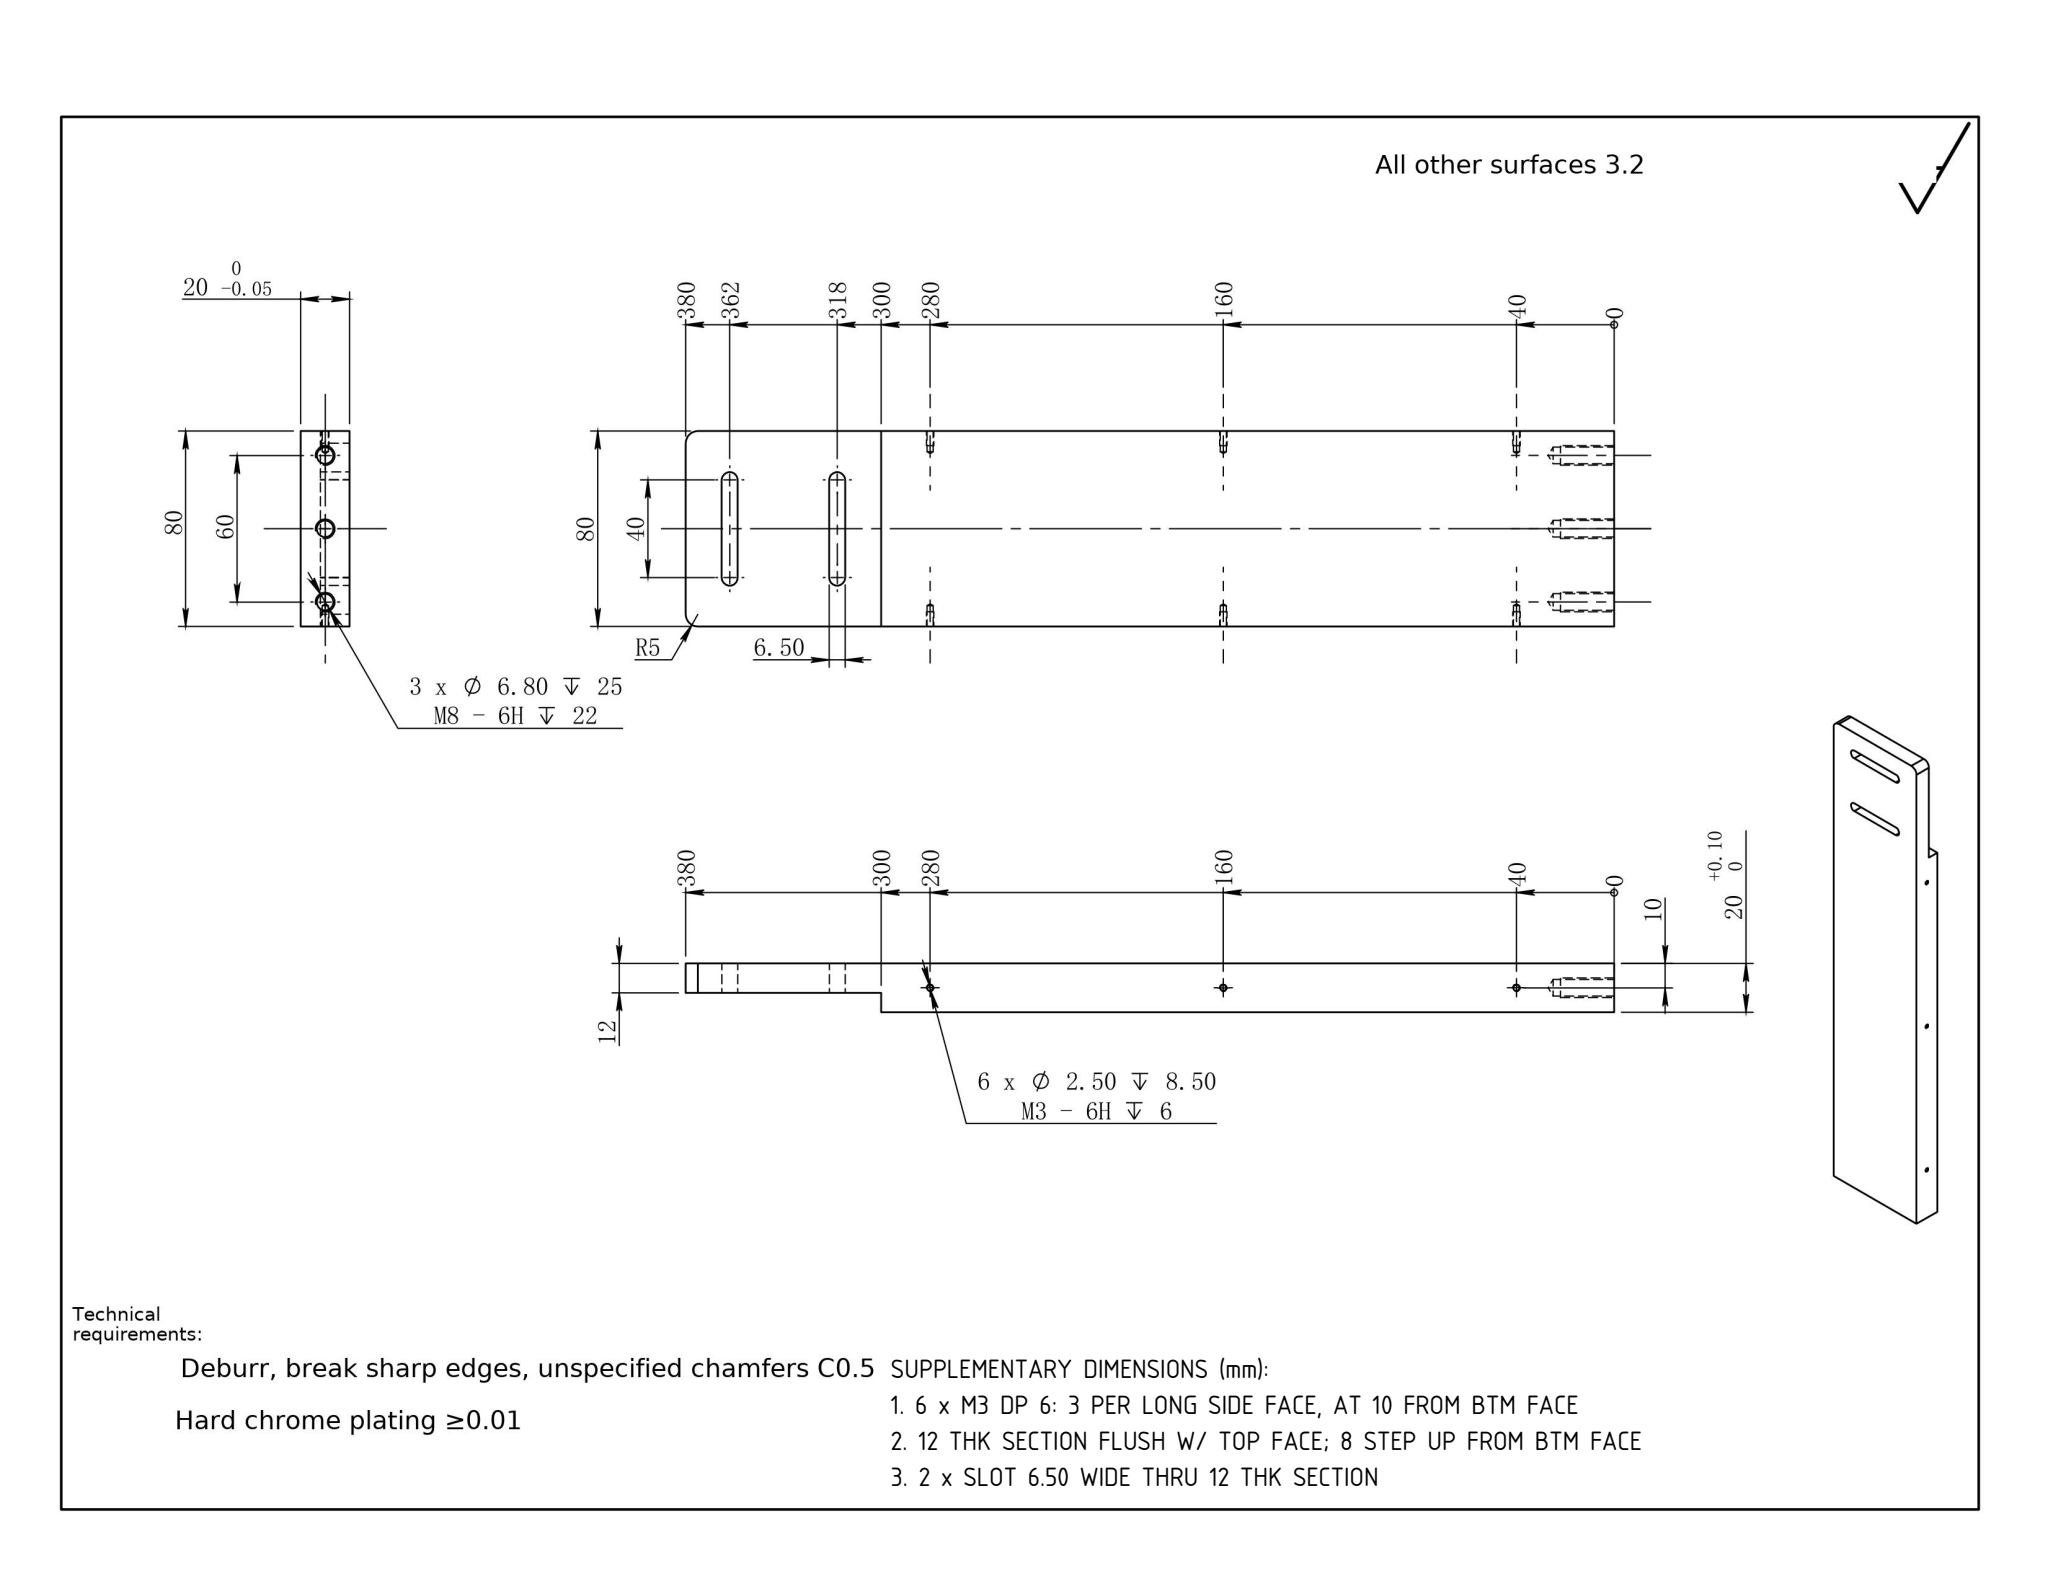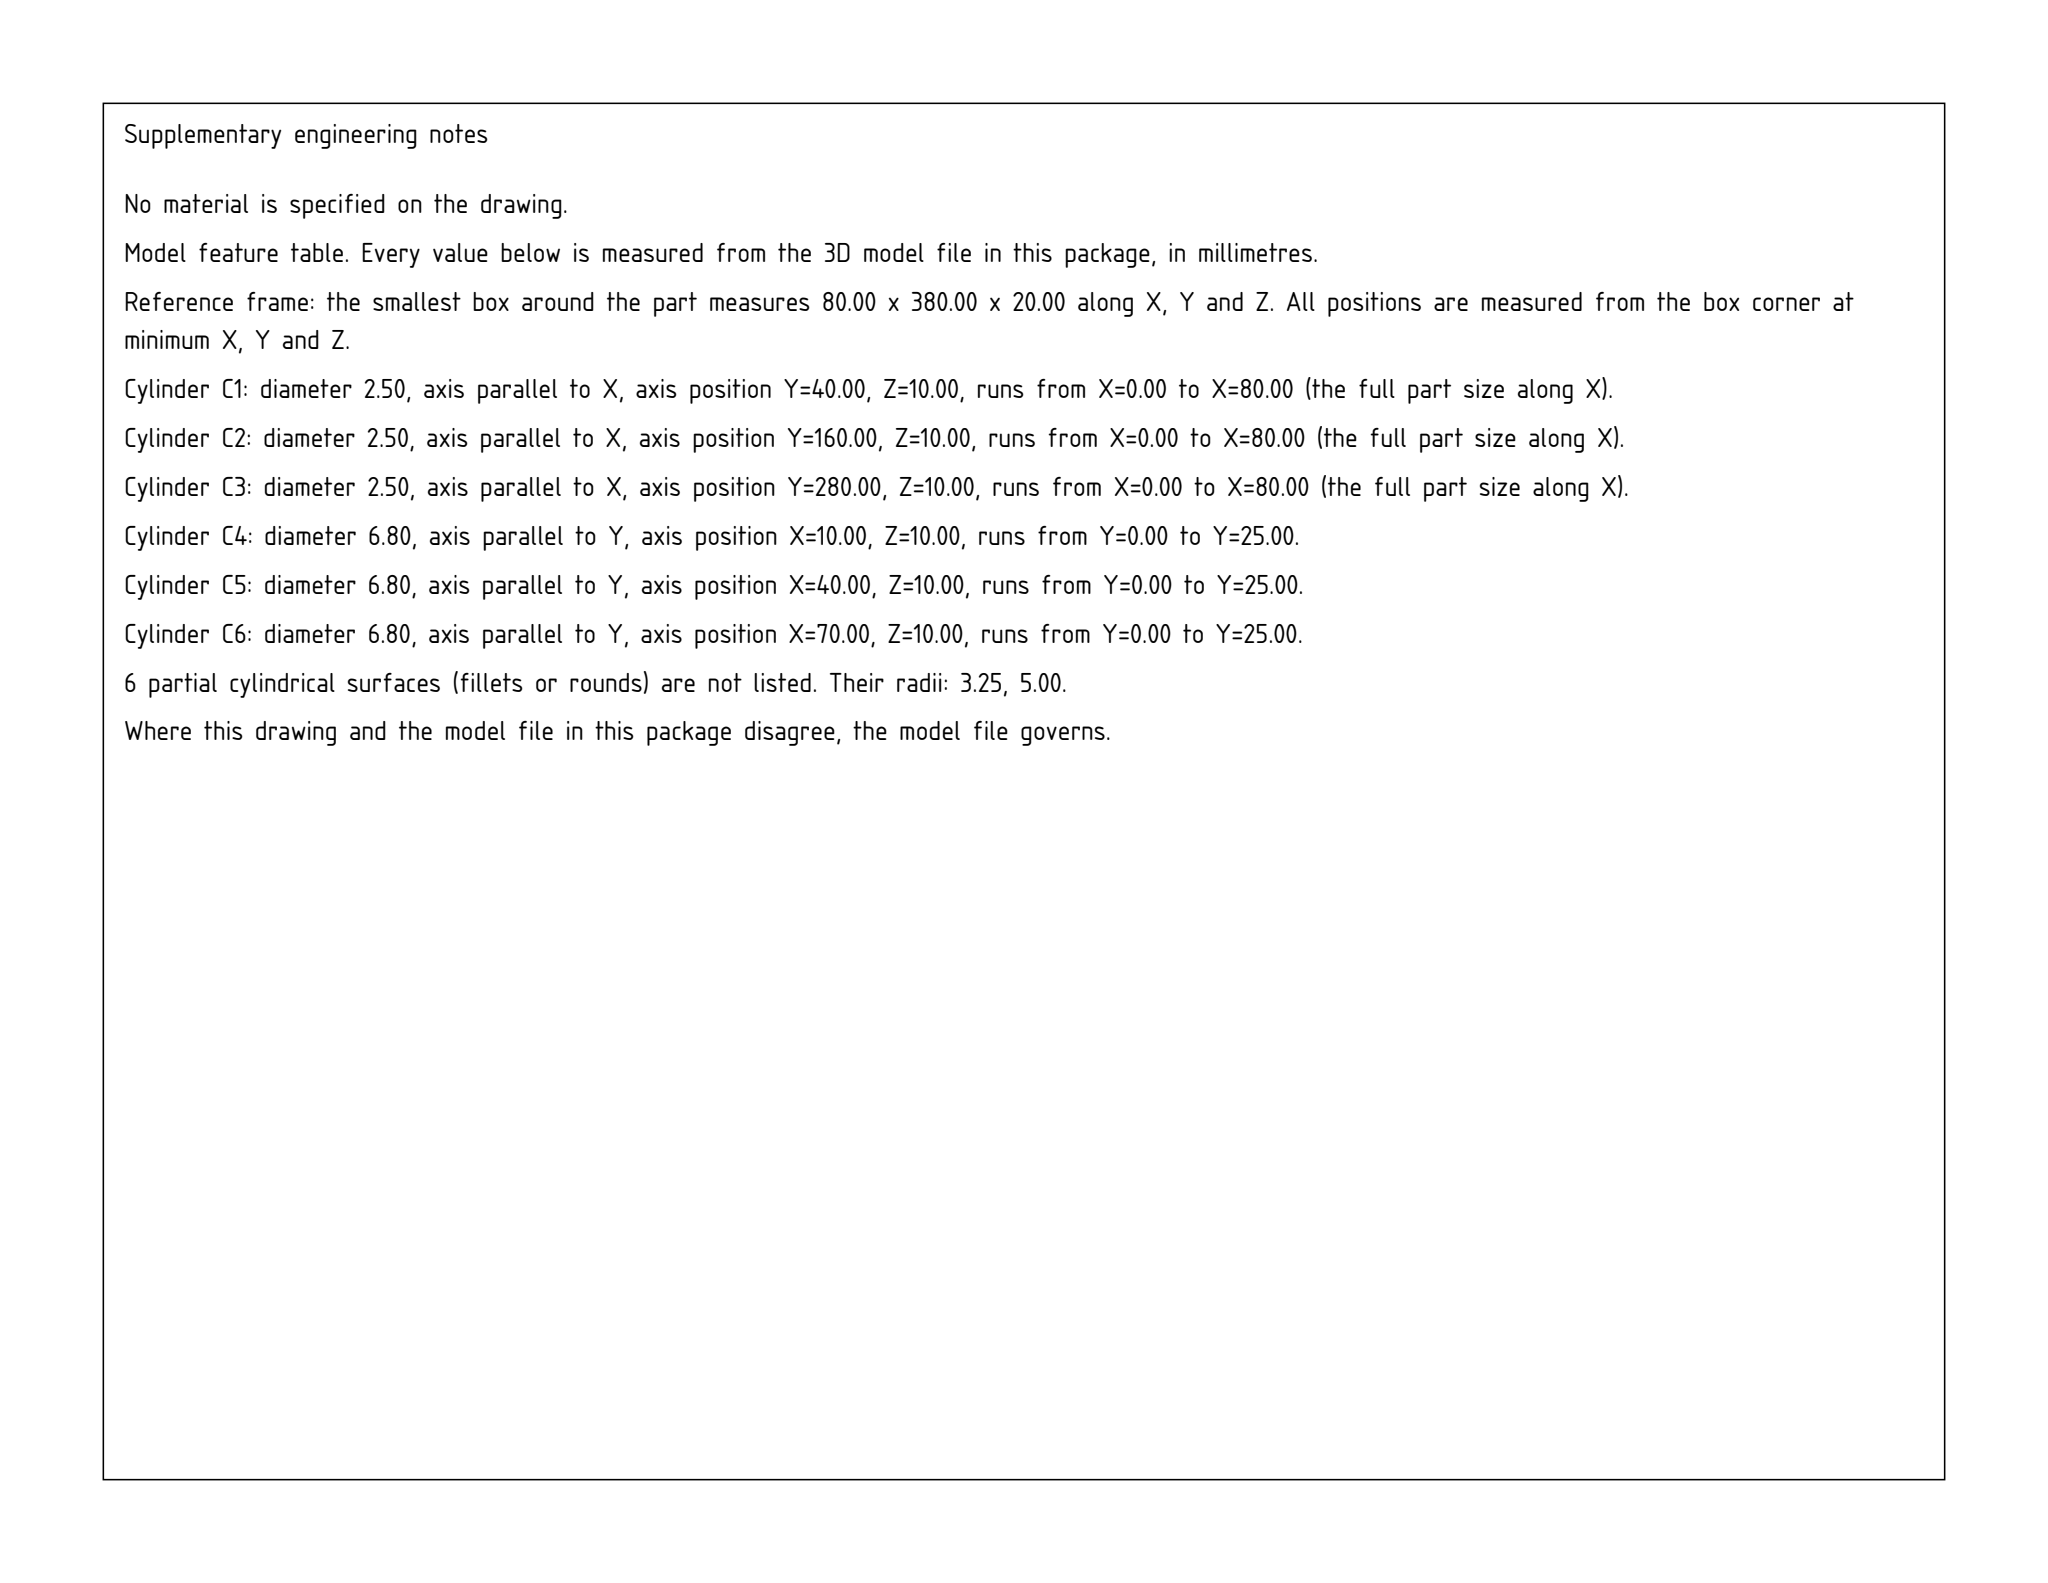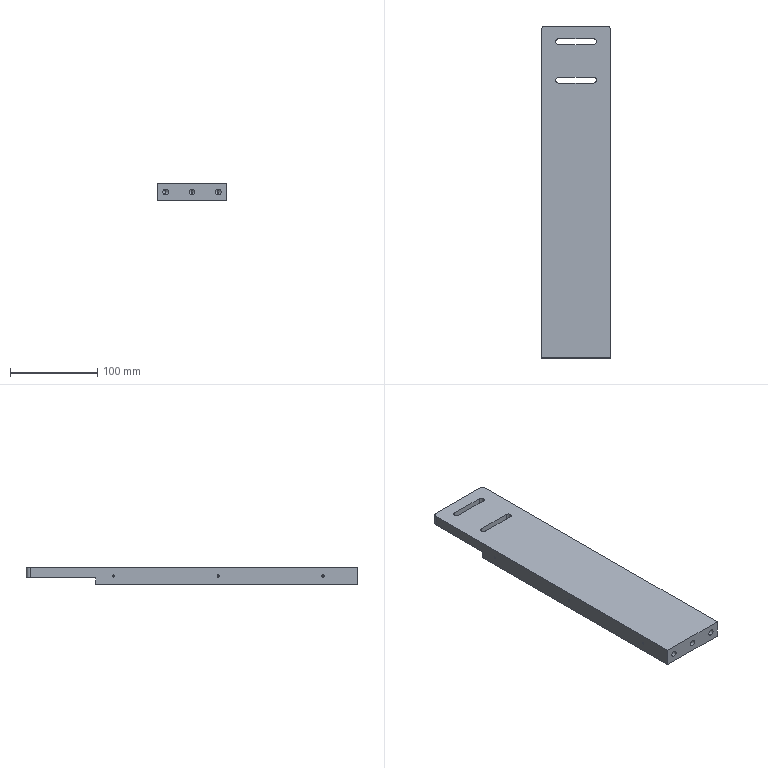Part | SolidWorks | mm | 1 solid | 56 faces | box 80 x 380 x 20 mm | volume 546579 mm3 | cylinder 26 | cone 18 | plane 12 | commonest cylinder face diameters 2.5 x12 6.5 x6 6.8 x6 10 x2
build123d program:
from build123d import *

# Parameters (mm, degrees)
SKETCH1_W             = 80
SKETCH1_H             = 380
BOSS_EXTRUDE1_DEPTH   = 10
M8_TAPPED_HOLE1_D     = 6.8
M8_TAPPED_HOLE1_DEPTH = 25
M8_TAPPED_HOLE1_TIP   = 2.043
CUT_EXTRUDE1_DEPTH    = 196.192
SKETCH8_W             = 8
SKETCH8_H             = 80
CUT_EXTRUDE2_DEPTH    = 207.398
LPATTERN1_COUNT       = 3
LPATTERN1_PITCH       = 120
FILLET1_R             = 5


with BuildPart() as part:
    # Sketch1 → Boss-Extrude1 (new, symmetric)
    with BuildSketch(Plane.XY):
        Rectangle(SKETCH1_W, SKETCH1_H)
    extrude(amount=BOSS_EXTRUDE1_DEPTH, both=True)

    # M8 Tapped Hole1
    with Locations(Plane(origin=(0, -190, 0), x_dir=(-1, 0, 0), z_dir=(0, -1, 0))):
        with Locations((30, 0), (-30, 0), (0, 0)):
            Hole(M8_TAPPED_HOLE1_D / 2, depth=M8_TAPPED_HOLE1_DEPTH)
            with Locations((0, 0, -(M8_TAPPED_HOLE1_DEPTH + M8_TAPPED_HOLE1_TIP / 2))):  # 118° drill point
                Cone(0, M8_TAPPED_HOLE1_D / 2, M8_TAPPED_HOLE1_TIP, mode=Mode.SUBTRACT)

    # Sketch7 → Cut-Extrude1 (cut, through all)
    with BuildSketch(Plane.XY.offset(10)):
        with BuildLine():
            Line((-20, 175.25), (20, 175.25))
            ThreePointArc((20, 175.25), (23.25, 172), (20, 168.75))
            Line((20, 168.75), (-20, 168.75))
            ThreePointArc((-20, 168.75), (-23.25, 172), (-20, 175.25))
        make_face()
        with BuildLine():
            Line((-20, 131.25), (20, 131.25))
            ThreePointArc((20, 131.25), (23.25, 128), (20, 124.75))
            Line((20, 124.75), (-20, 124.75))
            ThreePointArc((-20, 124.75), (-23.25, 128), (-20, 131.25))
        make_face()
    extrude(amount=-CUT_EXTRUDE1_DEPTH, mode=Mode.SUBTRACT)

    # Sketch8 → Cut-Extrude2 (cut, through all)
    with BuildSketch(Plane.ZY.offset(40)):
        with Locations((-6, 150)):
            Rectangle(SKETCH8_W, SKETCH8_H)
    extrude(amount=-CUT_EXTRUDE2_DEPTH, mode=Mode.SUBTRACT)

    # Sketch10 → M3 Tapped Hole1 (revolve, cut)
    with BuildSketch(Plane(origin=(-40, 90, 0), x_dir=(0, 0, 1), z_dir=(0, 1, 0))):
        Polygon((0, 0), (0, 9.251), (1.25, 8.5), (1.25, 0), align=None)
    m3_tapped_hole1 = revolve(axis=Axis((-46.35, 90, 0), (1, 0, 0)), mode=Mode.SUBTRACT)

    # LPattern1: M3 Tapped Hole1 ×3
    with Locations(*[(0, -i * LPATTERN1_PITCH, 0) for i in range(1, LPATTERN1_COUNT)]):
        add(m3_tapped_hole1, mode=Mode.SUBTRACT)

    # Mirror1: M3 Tapped Hole1 across plane
    add(m3_tapped_hole1.mirror(Plane(origin=(0, 0, 0), x_dir=(0, 0, 1), z_dir=(1, 0, 0))), mode=Mode.SUBTRACT)

    # Mirror1 copy 1 sketch → Mirror1 copy 1 (revolve, cut)
    with BuildSketch(Plane(origin=(40, -30, 0), x_dir=(0, 0, 1), z_dir=(0, 1, 0))):
        Polygon((0, 0), (0, -9.251), (1.25, -8.5), (1.25, 0), align=None)
    revolve(axis=Axis((46.35, -30, 0), (1, 0, 0)), mode=Mode.SUBTRACT)

    # Mirror1 copy 2 sketch → Mirror1 copy 2 (revolve, cut)
    with BuildSketch(Plane(origin=(40, -150, 0), x_dir=(0, 0, 1), z_dir=(0, 1, 0))):
        Polygon((0, 0), (0, -9.251), (1.25, -8.5), (1.25, 0), align=None)
    revolve(axis=Axis((46.35, -150, 0), (1, 0, 0)), mode=Mode.SUBTRACT)

    # Fillet1
    fillet1_edges = [part.edges().sort_by_distance(p)[0] for p in [
        (-40, 190, 4),
        (40, 190, 4),
    ]]
    fillet(fillet1_edges, radius=FILLET1_R)


solid = part.part